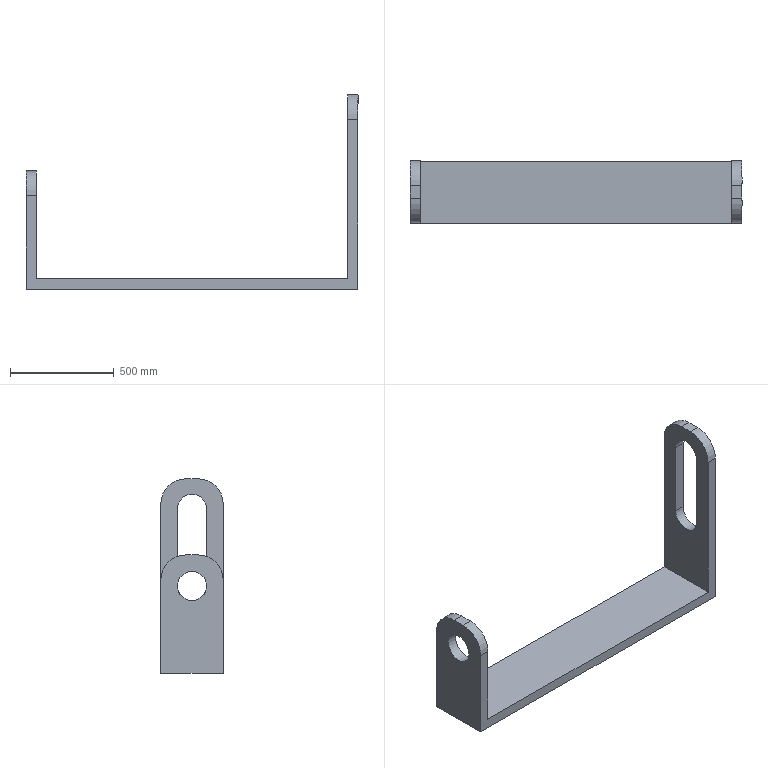Component | NX | MODEL82 | 1 solid | 19 faces | volume 40289242 mm3 | plane 12 | cylinder 7 | commonest cylinder face diameters 240 x4 141 x3